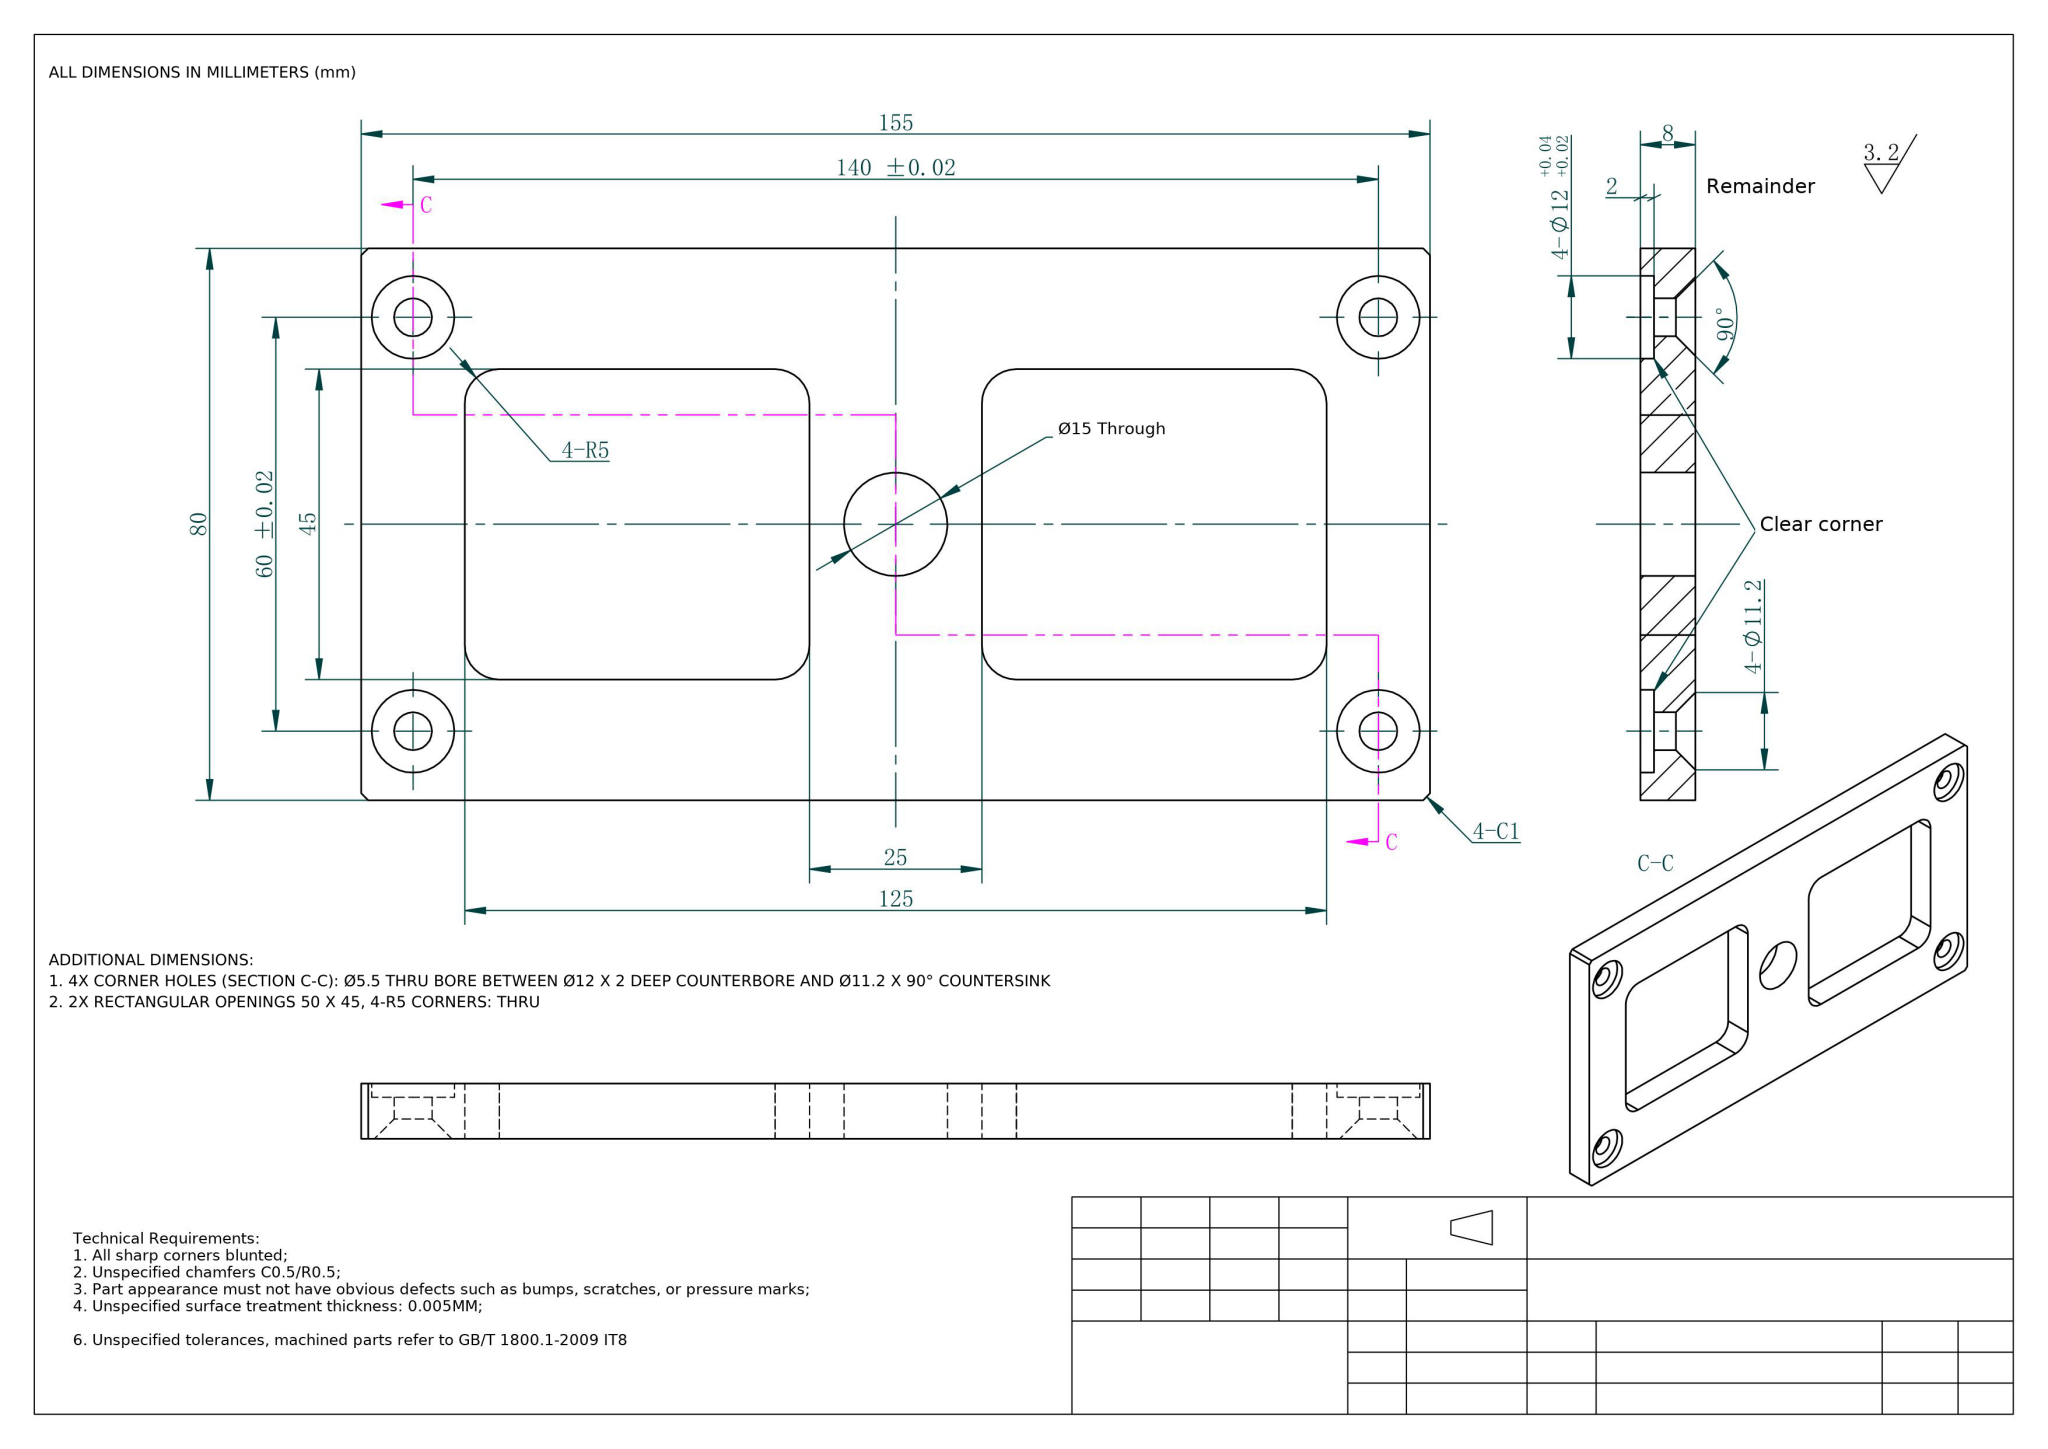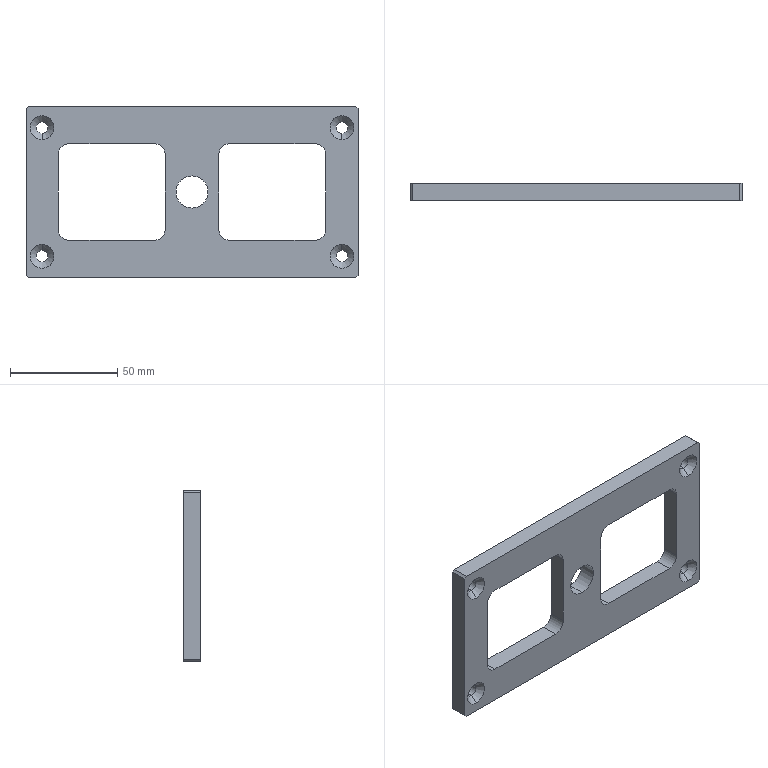Part | NX | mm | 1 solid | 56 faces | box 155 x 8 x 80 mm | volume 60261 mm3 | cylinder 26 | plane 22 | cone 8 | commonest cylinder face diameters 5.5 x8 12 x8 10 x8 15 x2